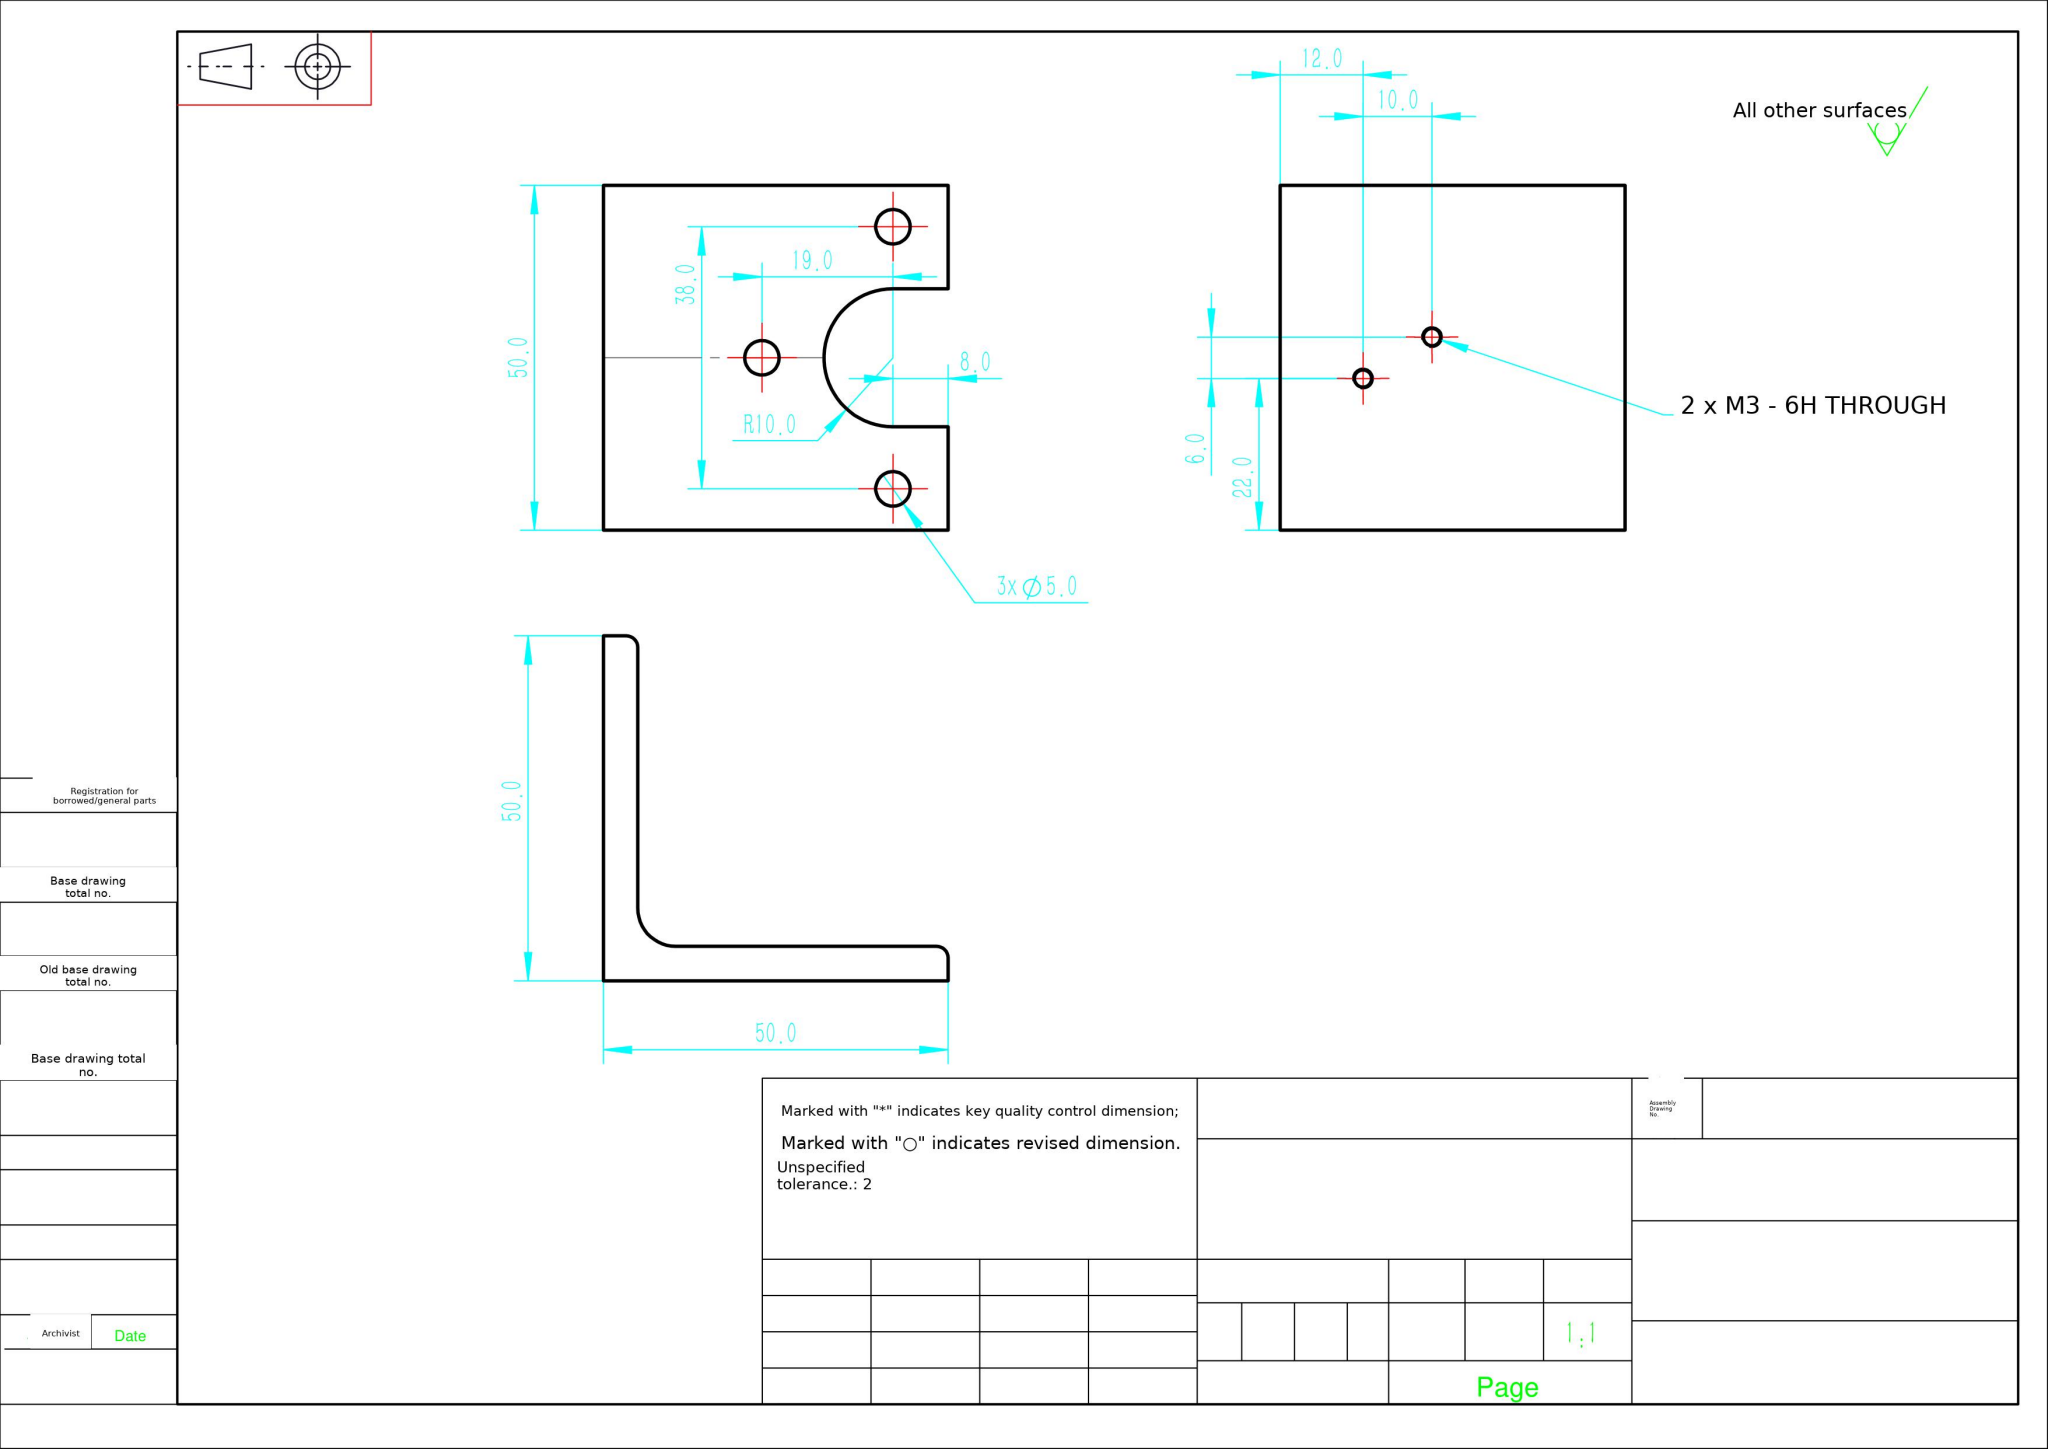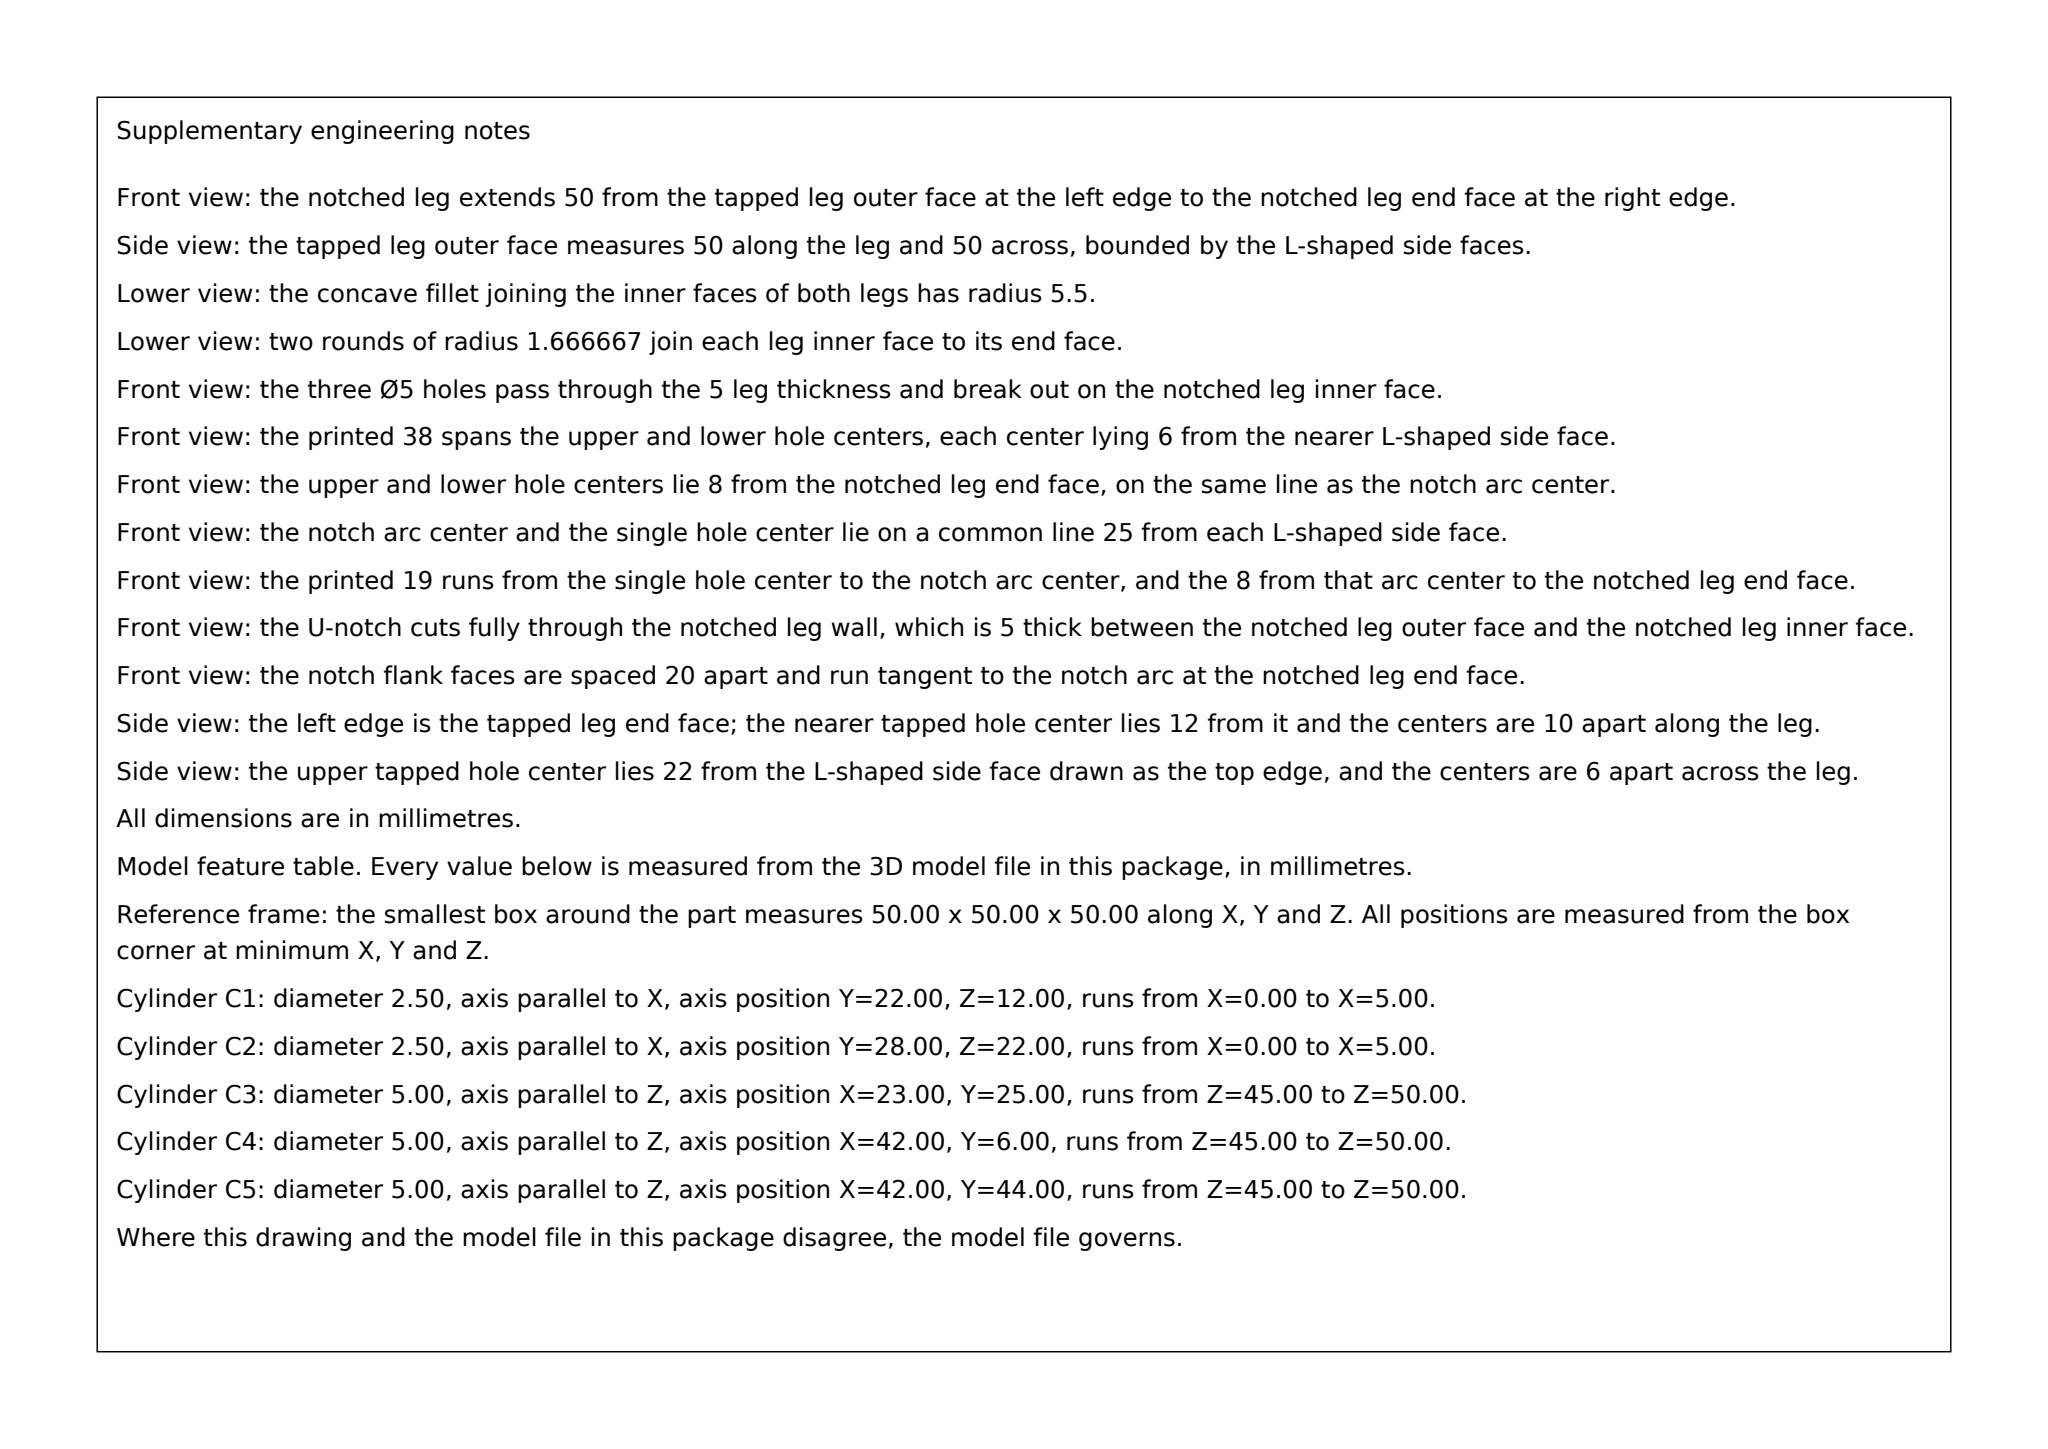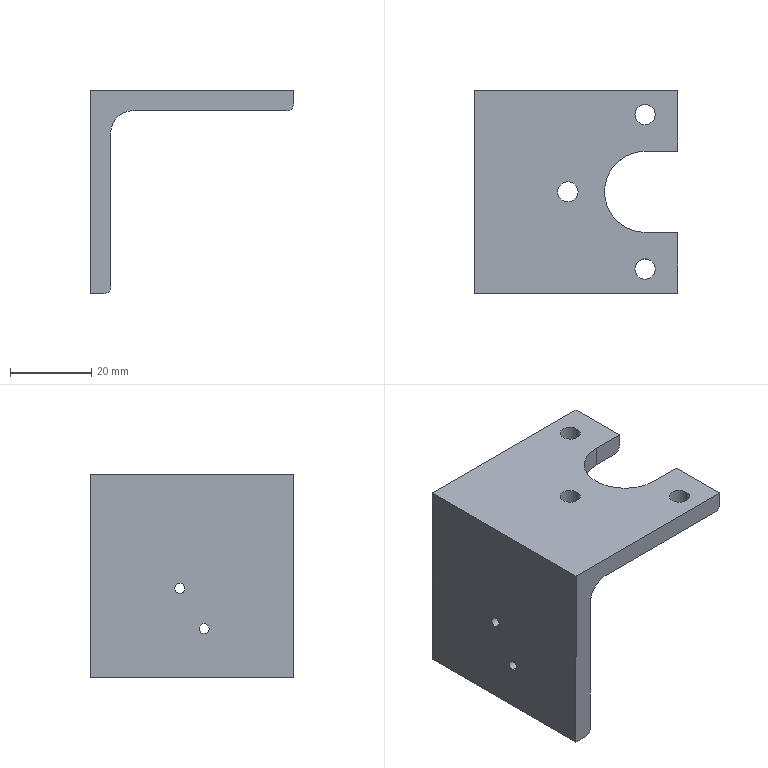Part | SolidWorks | mm | 1 solid | 26 faces | box 50 x 50 x 50 mm | volume 22098 mm3 | cylinder 15 | plane 11 | commonest cylinder face diameters 5 x6 2.5 x4 3.333 x3 11 x1 20 x1
Drawing notes:
HORIZ LEG THK 5.0 (SAME AS VERT LEG) | from the solid: Z planes at 45.0 and 50.0 with bbox Z=50; Ø5 holes axis z length 5.0
build123d program:
from build123d import *

# Parameters (mm, degrees)
STRUCTURAL_MEMBER1_DEPTH = 50
CUT_EXTRUDE1_REACH       = 66.413
SKETCH3_R                = 2.5
M3_TAPPED_HOLE1_D        = 2.5


with BuildPart() as part:
    # Sketch1 → Structural Member1 (new body)
    with BuildSketch(Plane(origin=(-32, -25, 0), x_dir=(1, 0, 0), z_dir=(0, -1, 0))):
        with BuildLine():
            Line((50, 0), (0, 0))
            Line((0, 0), (0, -50))
            Line((0, -50), (3.333, -50))
            ThreePointArc((3.333, -50), (4.512, -49.512), (5, -48.333))
            Line((5, -48.333), (5, -10.5))
            ThreePointArc((5, -10.5), (6.611, -6.611), (10.5, -5))
            Line((10.5, -5), (48.333, -5))
            ThreePointArc((48.333, -5), (49.512, -4.512), (50, -3.333))
            Line((50, -3.333), (50, 0))
        make_face()
    extrude(amount=-STRUCTURAL_MEMBER1_DEPTH)

    # Sketch3 → Cut-Extrude1 (cut, up to next)
    with BuildSketch(Plane.XY, mode=Mode.PRIVATE) as cut_extrude1_sk1:
        with Locations((10, -19)):
            Circle(SKETCH3_R)
    cut_extrude1_tool1 = extrude(cut_extrude1_sk1.sketch, amount=-CUT_EXTRUDE1_REACH, mode=Mode.PRIVATE) & part.part
    # Sketch3 → Cut-Extrude1 (cut, up to next)
    with BuildSketch(Plane.XY, mode=Mode.PRIVATE) as cut_extrude1_sk2:
        with Locations((-9, 0)):
            Circle(SKETCH3_R)
    cut_extrude1_tool2 = extrude(cut_extrude1_sk2.sketch, amount=-CUT_EXTRUDE1_REACH, mode=Mode.PRIVATE) & part.part
    # Sketch3 → Cut-Extrude1 (cut, up to next)
    with BuildSketch(Plane.XY, mode=Mode.PRIVATE) as cut_extrude1_sk3:
        with Locations((10, 19)):
            Circle(SKETCH3_R)
    cut_extrude1_tool3 = extrude(cut_extrude1_sk3.sketch, amount=-CUT_EXTRUDE1_REACH, mode=Mode.PRIVATE) & part.part
    # Sketch3 → Cut-Extrude1 (cut, up to next)
    with BuildSketch(Plane.XY, mode=Mode.PRIVATE) as cut_extrude1_sk4:
        with BuildLine():
            Line((10, 10), (18, 10))
            ThreePointArc((18, 10), (28, 0), (18, -10))
            Line((18, -10), (10, -10))
            ThreePointArc((10, -10), (0, 0), (10, 10))
        make_face()
    cut_extrude1_tool4 = extrude(cut_extrude1_sk4.sketch, amount=-CUT_EXTRUDE1_REACH, mode=Mode.PRIVATE) & part.part
    add(cut_extrude1_tool1.solids().sort_by_distance((10, -19, 0))[0], mode=Mode.SUBTRACT)
    add(cut_extrude1_tool2.solids().sort_by_distance((-9, 0, 0))[0], mode=Mode.SUBTRACT)
    add(cut_extrude1_tool3.solids().sort_by_distance((10, 19, 0))[0], mode=Mode.SUBTRACT)
    add(cut_extrude1_tool4.solids().sort_by_distance((14, 0, 0))[0], mode=Mode.SUBTRACT)

    # M3 Tapped Hole1 (through all)
    with Locations(Plane.ZY.offset(32)):
        with Locations((-28, 3), (-38, -3)):
            Hole(M3_TAPPED_HOLE1_D / 2)


solid = part.part
STEP:
#1=CARTESIAN_POINT('',(-27.,3.,-26.75));
#2=VERTEX_POINT('',#1);
#3=CARTESIAN_POINT('',(-27.,3.,-29.25));
#4=VERTEX_POINT('',#3);
#5=CARTESIAN_POINT('',(-27.,3.,-28.));
#6=DIRECTION('',(1.,0.,-0.));
#7=DIRECTION('',(-0.,0.,-1.));
#8=AXIS2_PLACEMENT_3D('',#5,#6,#7);
#9=CIRCLE('',#8,1.25);
#10=EDGE_CURVE('',#2,#4,#9,.T.);
#11=ORIENTED_EDGE('',*,*,#10,.T.);
#12=CARTESIAN_POINT('',(-32.,3.,-29.25));
#13=VERTEX_POINT('',#12);
#14=CARTESIAN_POINT('',(-32.,3.,-29.25));
#15=DIRECTION('',(-1.,0.,0.));
#16=VECTOR('',#15,1000.);
#17=LINE('',#14,#16);
#18=EDGE_CURVE('',#4,#13,#17,.T.);
#19=ORIENTED_EDGE('',*,*,#18,.T.);
#20=CARTESIAN_POINT('',(-32.,3.,-26.75));
#21=VERTEX_POINT('',#20);
#22=CARTESIAN_POINT('',(-32.,3.,-28.));
#23=DIRECTION('',(-1.,0.,0.));
#24=DIRECTION('',(0.,0.,1.));
#25=AXIS2_PLACEMENT_3D('',#22,#23,#24);
#26=CIRCLE('',#25,1.25);
#27=EDGE_CURVE('',#13,#21,#26,.T.);
#28=ORIENTED_EDGE('',*,*,#27,.T.);
#29=CARTESIAN_POINT('',(-32.,3.,-26.75));
#30=DIRECTION('',(-1.,0.,0.));
#31=VECTOR('',#30,1000.);
#32=LINE('',#29,#31);
#33=EDGE_CURVE('',#2,#21,#32,.T.);
#34=ORIENTED_EDGE('',*,*,#33,.F.);
#35=EDGE_LOOP('',(#11,#19,#28,#34));
#36=FACE_OUTER_BOUND('',#35,.T.);
#37=CARTESIAN_POINT('',(-32.,3.,-28.));
#38=DIRECTION('',(-1.,0.,0.));
#39=DIRECTION('',(0.,0.,1.));
#40=AXIS2_PLACEMENT_3D('',#37,#38,#39);
#41=CYLINDRICAL_SURFACE('',#40,1.25);
#42=ADVANCED_FACE('',(#36),#41,.F.);
#43=CARTESIAN_POINT('',(-27.,-3.,-36.75));
#44=VERTEX_POINT('',#43);
#45=CARTESIAN_POINT('',(-27.,-3.,-39.25));
#46=VERTEX_POINT('',#45);
#47=CARTESIAN_POINT('',(-27.,-3.,-38.));
#48=DIRECTION('',(1.,0.,-0.));
#49=DIRECTION('',(-0.,0.,-1.));
#50=AXIS2_PLACEMENT_3D('',#47,#48,#49);
#51=CIRCLE('',#50,1.25);
#52=EDGE_CURVE('',#44,#46,#51,.T.);
#53=ORIENTED_EDGE('',*,*,#52,.T.);
#54=CARTESIAN_POINT('',(-32.,-3.,-39.25));
#55=VERTEX_POINT('',#54);
#56=CARTESIAN_POINT('',(-32.,-3.,-39.25));
#57=DIRECTION('',(-1.,0.,0.));
#58=VECTOR('',#57,1000.);
#59=LINE('',#56,#58);
#60=EDGE_CURVE('',#46,#55,#59,.T.);
#61=ORIENTED_EDGE('',*,*,#60,.T.);
#62=CARTESIAN_POINT('',(-32.,-3.,-36.75));
#63=VERTEX_POINT('',#62);
#64=CARTESIAN_POINT('',(-32.,-3.,-38.));
#65=DIRECTION('',(-1.,0.,0.));
#66=DIRECTION('',(0.,0.,1.));
#67=AXIS2_PLACEMENT_3D('',#64,#65,#66);
#68=CIRCLE('',#67,1.25);
#69=EDGE_CURVE('',#55,#63,#68,.T.);
#70=ORIENTED_EDGE('',*,*,#69,.T.);
#71=CARTESIAN_POINT('',(-32.,-3.,-36.75));
#72=DIRECTION('',(-1.,0.,0.));
#73=VECTOR('',#72,1000.);
#74=LINE('',#71,#73);
#75=EDGE_CURVE('',#44,#63,#74,.T.);
#76=ORIENTED_EDGE('',*,*,#75,.F.);
#77=EDGE_LOOP('',(#53,#61,#70,#76));
#78=FACE_OUTER_BOUND('',#77,.T.);
#79=CARTESIAN_POINT('',(-32.,-3.,-38.));
#80=DIRECTION('',(-1.,0.,0.));
#81=DIRECTION('',(0.,0.,1.));
#82=AXIS2_PLACEMENT_3D('',#79,#80,#81);
#83=CYLINDRICAL_SURFACE('',#82,1.25);
#84=ADVANCED_FACE('',(#78),#83,.F.);
#85=CARTESIAN_POINT('',(7.5,19.,-5.));
#86=VERTEX_POINT('',#85);
#87=CARTESIAN_POINT('',(12.5,19.,-5.));
#88=VERTEX_POINT('',#87);
#89=CARTESIAN_POINT('',(10.,19.,-5.));
#90=DIRECTION('',(0.,0.,1.));
#91=DIRECTION('',(-1.,0.,0.));
#92=AXIS2_PLACEMENT_3D('',#89,#90,#91);
#93=CIRCLE('',#92,2.5);
#94=EDGE_CURVE('',#86,#88,#93,.T.);
#95=ORIENTED_EDGE('',*,*,#94,.F.);
#96=CARTESIAN_POINT('',(7.5,19.,0.));
#97=VERTEX_POINT('',#96);
#98=CARTESIAN_POINT('',(7.5,19.,-50.001));
#99=DIRECTION('',(0.,0.,1.));
#100=VECTOR('',#99,1000.);
#101=LINE('',#98,#100);
#102=EDGE_CURVE('',#86,#97,#101,.T.);
#103=ORIENTED_EDGE('',*,*,#102,.T.);
#104=CARTESIAN_POINT('',(12.5,19.,0.));
#105=VERTEX_POINT('',#104);
#106=CARTESIAN_POINT('',(10.,19.,0.));
#107=DIRECTION('',(0.,0.,1.));
#108=DIRECTION('',(1.,0.,0.));
#109=AXIS2_PLACEMENT_3D('',#106,#107,#108);
#110=CIRCLE('',#109,2.5);
#111=EDGE_CURVE('',#97,#105,#110,.T.);
#112=ORIENTED_EDGE('',*,*,#111,.T.);
#113=CARTESIAN_POINT('',(12.5,19.,-50.001));
#114=DIRECTION('',(0.,0.,1.));
#115=VECTOR('',#114,1000.);
#116=LINE('',#113,#115);
#117=EDGE_CURVE('',#88,#105,#116,.T.);
#118=ORIENTED_EDGE('',*,*,#117,.F.);
#119=EDGE_LOOP('',(#95,#103,#112,#118));
#120=FACE_OUTER_BOUND('',#119,.T.);
#121=CARTESIAN_POINT('',(10.,19.,-50.001));
#122=DIRECTION('',(0.,0.,1.));
#123=DIRECTION('',(1.,0.,0.));
#124=AXIS2_PLACEMENT_3D('',#121,#122,#123);
#125=CYLINDRICAL_SURFACE('',#124,2.5);
#126=ADVANCED_FACE('',(#120),#125,.F.);
#127=CARTESIAN_POINT('',(-11.5,-0.,-5.));
#128=VERTEX_POINT('',#127);
#129=CARTESIAN_POINT('',(-6.5,-0.,-5.));
#130=VERTEX_POINT('',#129);
#131=CARTESIAN_POINT('',(-9.,-0.,-5.));
#132=DIRECTION('',(0.,0.,1.));
#133=DIRECTION('',(-1.,0.,0.));
#134=AXIS2_PLACEMENT_3D('',#131,#132,#133);
#135=CIRCLE('',#134,2.5);
#136=EDGE_CURVE('',#128,#130,#135,.T.);
#137=ORIENTED_EDGE('',*,*,#136,.F.);
#138=CARTESIAN_POINT('',(-11.5,-0.,0.));
#139=VERTEX_POINT('',#138);
#140=CARTESIAN_POINT('',(-11.5,-0.,-50.001));
#141=DIRECTION('',(0.,0.,1.));
#142=VECTOR('',#141,1000.);
#143=LINE('',#140,#142);
#144=EDGE_CURVE('',#128,#139,#143,.T.);
#145=ORIENTED_EDGE('',*,*,#144,.T.);
#146=CARTESIAN_POINT('',(-6.5,-0.,0.));
#147=VERTEX_POINT('',#146);
#148=CARTESIAN_POINT('',(-9.,-0.,0.));
#149=DIRECTION('',(0.,0.,1.));
#150=DIRECTION('',(1.,0.,0.));
#151=AXIS2_PLACEMENT_3D('',#148,#149,#150);
#152=CIRCLE('',#151,2.5);
#153=EDGE_CURVE('',#139,#147,#152,.T.);
#154=ORIENTED_EDGE('',*,*,#153,.T.);
#155=CARTESIAN_POINT('',(-6.5,-0.,-50.001));
#156=DIRECTION('',(0.,0.,1.));
#157=VECTOR('',#156,1000.);
#158=LINE('',#155,#157);
#159=EDGE_CURVE('',#130,#147,#158,.T.);
#160=ORIENTED_EDGE('',*,*,#159,.F.);
#161=EDGE_LOOP('',(#137,#145,#154,#160));
#162=FACE_OUTER_BOUND('',#161,.T.);
#163=CARTESIAN_POINT('',(-9.,-0.,-50.001));
#164=DIRECTION('',(0.,0.,1.));
#165=DIRECTION('',(1.,0.,0.));
#166=AXIS2_PLACEMENT_3D('',#163,#164,#165);
#167=CYLINDRICAL_SURFACE('',#166,2.5);
#168=ADVANCED_FACE('',(#162),#167,.F.);
#169=CARTESIAN_POINT('',(7.5,-19.,-5.));
#170=VERTEX_POINT('',#169);
#171=CARTESIAN_POINT('',(12.5,-19.,-5.));
#172=VERTEX_POINT('',#171);
#173=CARTESIAN_POINT('',(10.,-19.,-5.));
#174=DIRECTION('',(0.,0.,1.));
#175=DIRECTION('',(-1.,0.,0.));
#176=AXIS2_PLACEMENT_3D('',#173,#174,#175);
#177=CIRCLE('',#176,2.5);
#178=EDGE_CURVE('',#170,#172,#177,.T.);
#179=ORIENTED_EDGE('',*,*,#178,.F.);
#180=CARTESIAN_POINT('',(7.5,-19.,0.));
#181=VERTEX_POINT('',#180);
#182=CARTESIAN_POINT('',(7.5,-19.,-50.001));
#183=DIRECTION('',(0.,0.,1.));
#184=VECTOR('',#183,1000.);
#185=LINE('',#182,#184);
#186=EDGE_CURVE('',#170,#181,#185,.T.);
#187=ORIENTED_EDGE('',*,*,#186,.T.);
#188=CARTESIAN_POINT('',(12.5,-19.,0.));
#189=VERTEX_POINT('',#188);
#190=CARTESIAN_POINT('',(10.,-19.,0.));
#191=DIRECTION('',(0.,0.,1.));
#192=DIRECTION('',(1.,0.,0.));
#193=AXIS2_PLACEMENT_3D('',#190,#191,#192);
#194=CIRCLE('',#193,2.5);
#195=EDGE_CURVE('',#181,#189,#194,.T.);
#196=ORIENTED_EDGE('',*,*,#195,.T.);
#197=CARTESIAN_POINT('',(12.5,-19.,-50.001));
#198=DIRECTION('',(0.,0.,1.));
#199=VECTOR('',#198,1000.);
#200=LINE('',#197,#199);
#201=EDGE_CURVE('',#172,#189,#200,.T.);
#202=ORIENTED_EDGE('',*,*,#201,.F.);
#203=EDGE_LOOP('',(#179,#187,#196,#202));
#204=FACE_OUTER_BOUND('',#203,.T.);
#205=CARTESIAN_POINT('',(10.,-19.,-50.001));
#206=DIRECTION('',(0.,0.,1.));
#207=DIRECTION('',(1.,0.,0.));
#208=AXIS2_PLACEMENT_3D('',#205,#206,#207);
#209=CYLINDRICAL_SURFACE('',#208,2.5);
#210=ADVANCED_FACE('',(#204),#209,.F.);
#211=CARTESIAN_POINT('',(18.,10.,0.));
#212=VERTEX_POINT('',#211);
#213=CARTESIAN_POINT('',(18.,10.,-3.333));
#214=VERTEX_POINT('',#213);
#215=CARTESIAN_POINT('',(18.,10.,-50.001));
#216=DIRECTION('',(0.,0.,-1.));
#217=VECTOR('',#216,1000.);
#218=LINE('',#215,#217);
#219=EDGE_CURVE('',#212,#214,#218,.T.);
#220=ORIENTED_EDGE('',*,*,#219,.T.);
#221=CARTESIAN_POINT('',(18.,25.,-3.333));
#222=VERTEX_POINT('',#221);
#223=CARTESIAN_POINT('',(18.,25.,-3.333));
#224=DIRECTION('',(0.,-1.,0.));
#225=VECTOR('',#224,1000.);
#226=LINE('',#223,#225);
#227=EDGE_CURVE('',#222,#214,#226,.T.);
#228=ORIENTED_EDGE('',*,*,#227,.F.);
#229=CARTESIAN_POINT('',(18.,25.,-0.));
#230=VERTEX_POINT('',#229);
#231=CARTESIAN_POINT('',(18.,25.,-0.));
#232=DIRECTION('',(0.,-0.,1.));
#233=VECTOR('',#232,1000.);
#234=LINE('',#231,#233);
#235=EDGE_CURVE('',#222,#230,#234,.T.);
#236=ORIENTED_EDGE('',*,*,#235,.T.);
#237=CARTESIAN_POINT('',(18.,25.,-0.));
#238=DIRECTION('',(0.,-1.,0.));
#239=VECTOR('',#238,1000.);
#240=LINE('',#237,#239);
#241=EDGE_CURVE('',#230,#212,#240,.T.);
#242=ORIENTED_EDGE('',*,*,#241,.T.);
#243=EDGE_LOOP('',(#220,#228,#236,#242));
#244=FACE_OUTER_BOUND('',#243,.T.);
#245=CARTESIAN_POINT('',(18.,25.,-0.));
#246=DIRECTION('',(1.,0.,-0.));
#247=DIRECTION('',(-0.,0.,-1.));
#248=AXIS2_PLACEMENT_3D('',#245,#246,#247);
#249=PLANE('',#248);
#250=ADVANCED_FACE('',(#244),#249,.T.);
#251=CARTESIAN_POINT('',(16.333,10.,-5.));
#252=VERTEX_POINT('',#251);
#253=CARTESIAN_POINT('',(16.333,10.,-3.333));
#254=DIRECTION('',(0.,1.,0.));
#255=DIRECTION('',(0.,0.,1.));
#256=AXIS2_PLACEMENT_3D('',#253,#254,#255);
#257=CIRCLE('',#256,1.667);
#258=EDGE_CURVE('',#214,#252,#257,.T.);
#259=ORIENTED_EDGE('',*,*,#258,.T.);
#260=CARTESIAN_POINT('',(16.333,25.,-5.));
#261=VERTEX_POINT('',#260);
#262=CARTESIAN_POINT('',(16.333,25.,-5.));
#263=DIRECTION('',(0.,-1.,0.));
#264=VECTOR('',#263,1000.);
#265=LINE('',#262,#264);
#266=EDGE_CURVE('',#261,#252,#265,.T.);
#267=ORIENTED_EDGE('',*,*,#266,.F.);
#268=CARTESIAN_POINT('',(16.333,25.,-3.333));
#269=DIRECTION('',(-0.,-1.,-0.));
#270=DIRECTION('',(-0.,0.,-1.));
#271=AXIS2_PLACEMENT_3D('',#268,#269,#270);
#272=CIRCLE('',#271,1.667);
#273=EDGE_CURVE('',#261,#222,#272,.T.);
#274=ORIENTED_EDGE('',*,*,#273,.T.);
#275=ORIENTED_EDGE('',*,*,#227,.T.);
#276=EDGE_LOOP('',(#259,#267,#274,#275));
#277=FACE_OUTER_BOUND('',#276,.T.);
#278=CARTESIAN_POINT('',(16.333,25.,-3.333));
#279=DIRECTION('',(0.,-1.,0.));
#280=DIRECTION('',(0.,0.,-1.));
#281=AXIS2_PLACEMENT_3D('',#278,#279,#280);
#282=CYLINDRICAL_SURFACE('',#281,1.667);
#283=ADVANCED_FACE('',(#277),#282,.T.);
#284=CARTESIAN_POINT('',(18.,-10.,-3.333));
#285=VERTEX_POINT('',#284);
#286=CARTESIAN_POINT('',(18.,-10.,-0.));
#287=VERTEX_POINT('',#286);
#288=CARTESIAN_POINT('',(18.,-10.,-50.001));
#289=DIRECTION('',(0.,0.,1.));
#290=VECTOR('',#289,1000.);
#291=LINE('',#288,#290);
#292=EDGE_CURVE('',#285,#287,#291,.T.);
#293=ORIENTED_EDGE('',*,*,#292,.T.);
#294=CARTESIAN_POINT('',(18.,-25.,-0.));
#295=VERTEX_POINT('',#294);
#296=CARTESIAN_POINT('',(18.,25.,-0.));
#297=DIRECTION('',(0.,-1.,0.));
#298=VECTOR('',#297,1000.);
#299=LINE('',#296,#298);
#300=EDGE_CURVE('',#287,#295,#299,.T.);
#301=ORIENTED_EDGE('',*,*,#300,.T.);
#302=CARTESIAN_POINT('',(18.,-25.,-3.333));
#303=VERTEX_POINT('',#302);
#304=CARTESIAN_POINT('',(18.,-25.,-0.));
#305=DIRECTION('',(0.,-0.,1.));
#306=VECTOR('',#305,1000.);
#307=LINE('',#304,#306);
#308=EDGE_CURVE('',#303,#295,#307,.T.);
#309=ORIENTED_EDGE('',*,*,#308,.F.);
#310=CARTESIAN_POINT('',(18.,25.,-3.333));
#311=DIRECTION('',(0.,-1.,0.));
#312=VECTOR('',#311,1000.);
#313=LINE('',#310,#312);
#314=EDGE_CURVE('',#285,#303,#313,.T.);
#315=ORIENTED_EDGE('',*,*,#314,.F.);
#316=EDGE_LOOP('',(#293,#301,#309,#315));
#317=FACE_OUTER_BOUND('',#316,.T.);
#318=CARTESIAN_POINT('',(18.,25.,-0.));
#319=DIRECTION('',(1.,0.,-0.));
#320=DIRECTION('',(-0.,0.,-1.));
#321=AXIS2_PLACEMENT_3D('',#318,#319,#320);
#322=PLANE('',#321);
#323=ADVANCED_FACE('',(#317),#322,.T.);
#324=CARTESIAN_POINT('',(16.333,-10.,-5.));
#325=VERTEX_POINT('',#324);
#326=CARTESIAN_POINT('',(16.333,-10.,-3.333));
#327=DIRECTION('',(0.,-1.,0.));
#328=DIRECTION('',(0.,0.,-1.));
#329=AXIS2_PLACEMENT_3D('',#326,#327,#328);
#330=CIRCLE('',#329,1.667);
#331=EDGE_CURVE('',#325,#285,#330,.T.);
#332=ORIENTED_EDGE('',*,*,#331,.T.);
#333=ORIENTED_EDGE('',*,*,#314,.T.);
#334=CARTESIAN_POINT('',(16.333,-25.,-5.));
#335=VERTEX_POINT('',#334);
#336=CARTESIAN_POINT('',(16.333,-25.,-3.333));
#337=DIRECTION('',(-0.,-1.,-0.));
#338=DIRECTION('',(-0.,0.,-1.));
#339=AXIS2_PLACEMENT_3D('',#336,#337,#338);
#340=CIRCLE('',#339,1.667);
#341=EDGE_CURVE('',#335,#303,#340,.T.);
#342=ORIENTED_EDGE('',*,*,#341,.F.);
#343=CARTESIAN_POINT('',(16.333,25.,-5.));
#344=DIRECTION('',(0.,-1.,0.));
#345=VECTOR('',#344,1000.);
#346=LINE('',#343,#345);
#347=EDGE_CURVE('',#325,#335,#346,.T.);
#348=ORIENTED_EDGE('',*,*,#347,.F.);
#349=EDGE_LOOP('',(#332,#333,#342,#348));
#350=FACE_OUTER_BOUND('',#349,.T.);
#351=CARTESIAN_POINT('',(16.333,25.,-3.333));
#352=DIRECTION('',(0.,-1.,0.));
#353=DIRECTION('',(0.,0.,-1.));
#354=AXIS2_PLACEMENT_3D('',#351,#352,#353);
#355=CYLINDRICAL_SURFACE('',#354,1.667);
#356=ADVANCED_FACE('',(#350),#355,.T.);
#357=CARTESIAN_POINT('',(10.,19.,-5.));
#358=DIRECTION('',(0.,0.,1.));
#359=DIRECTION('',(-1.,0.,0.));
#360=AXIS2_PLACEMENT_3D('',#357,#358,#359);
#361=CIRCLE('',#360,2.5);
#362=EDGE_CURVE('',#88,#86,#361,.T.);
#363=ORIENTED_EDGE('',*,*,#362,.T.);
#364=ORIENTED_EDGE('',*,*,#94,.T.);
#365=EDGE_LOOP('',(#363,#364));
#366=FACE_BOUND('',#365,.T.);
#367=CARTESIAN_POINT('',(10.,10.,-5.));
#368=VERTEX_POINT('',#367);
#369=CARTESIAN_POINT('',(10.,10.,-5.));
#370=DIRECTION('',(-1.,0.,0.));
#371=VECTOR('',#370,1000.);
#372=LINE('',#369,#371);
#373=EDGE_CURVE('',#252,#368,#372,.T.);
#374=ORIENTED_EDGE('',*,*,#373,.T.);
#375=CARTESIAN_POINT('',(10.,-10.,-5.));
#376=VERTEX_POINT('',#375);
#377=CARTESIAN_POINT('',(10.,-0.,-5.));
#378=DIRECTION('',(0.,0.,1.));
#379=DIRECTION('',(-1.,0.,0.));
#380=AXIS2_PLACEMENT_3D('',#377,#378,#379);
#381=CIRCLE('',#380,10.);
#382=EDGE_CURVE('',#368,#376,#381,.T.);
#383=ORIENTED_EDGE('',*,*,#382,.T.);
#384=CARTESIAN_POINT('',(10.,-10.,-5.));
#385=DIRECTION('',(1.,0.,-0.));
#386=VECTOR('',#385,1000.);
#387=LINE('',#384,#386);
#388=EDGE_CURVE('',#376,#325,#387,.T.);
#389=ORIENTED_EDGE('',*,*,#388,.T.);
#390=ORIENTED_EDGE('',*,*,#347,.T.);
#391=CARTESIAN_POINT('',(-21.5,-25.,-5.));
#392=VERTEX_POINT('',#391);
#393=CARTESIAN_POINT('',(16.333,-25.,-5.));
#394=DIRECTION('',(1.,-0.,-0.));
#395=VECTOR('',#394,1000.);
#396=LINE('',#393,#395);
#397=EDGE_CURVE('',#392,#335,#396,.T.);
#398=ORIENTED_EDGE('',*,*,#397,.F.);
#399=CARTESIAN_POINT('',(-21.5,25.,-5.));
#400=VERTEX_POINT('',#399);
#401=CARTESIAN_POINT('',(-21.5,25.,-5.));
#402=DIRECTION('',(0.,-1.,0.));
#403=VECTOR('',#402,1000.);
#404=LINE('',#401,#403);
#405=EDGE_CURVE('',#400,#392,#404,.T.);
#406=ORIENTED_EDGE('',*,*,#405,.F.);
#407=CARTESIAN_POINT('',(16.333,25.,-5.));
#408=DIRECTION('',(1.,-0.,-0.));
#409=VECTOR('',#408,1000.);
#410=LINE('',#407,#409);
#411=EDGE_CURVE('',#400,#261,#410,.T.);
#412=ORIENTED_EDGE('',*,*,#411,.T.);
#413=ORIENTED_EDGE('',*,*,#266,.T.);
#414=EDGE_LOOP('',(#374,#383,#389,#390,#398,#406,#412,#413));
#415=FACE_OUTER_BOUND('',#414,.T.);
#416=CARTESIAN_POINT('',(-9.,-0.,-5.));
#417=DIRECTION('',(0.,0.,1.));
#418=DIRECTION('',(-1.,0.,0.));
#419=AXIS2_PLACEMENT_3D('',#416,#417,#418);
#420=CIRCLE('',#419,2.5);
#421=EDGE_CURVE('',#130,#128,#420,.T.);
#422=ORIENTED_EDGE('',*,*,#421,.T.);
#423=ORIENTED_EDGE('',*,*,#136,.T.);
#424=EDGE_LOOP('',(#422,#423));
#425=FACE_BOUND('',#424,.T.);
#426=CARTESIAN_POINT('',(10.,-19.,-5.));
#427=DIRECTION('',(0.,0.,1.));
#428=DIRECTION('',(-1.,0.,0.));
#429=AXIS2_PLACEMENT_3D('',#426,#427,#428);
#430=CIRCLE('',#429,2.5);
#431=EDGE_CURVE('',#172,#170,#430,.T.);
#432=ORIENTED_EDGE('',*,*,#431,.T.);
#433=ORIENTED_EDGE('',*,*,#178,.T.);
#434=EDGE_LOOP('',(#432,#433));
#435=FACE_BOUND('',#434,.T.);
#436=CARTESIAN_POINT('',(16.333,25.,-5.));
#437=DIRECTION('',(-0.,0.,-1.));
#438=DIRECTION('',(-1.,0.,0.));
#439=AXIS2_PLACEMENT_3D('',#436,#437,#438);
#440=PLANE('',#439);
#441=ADVANCED_FACE('',(#366,#415,#425,#435),#440,.T.);
#442=CARTESIAN_POINT('',(-27.,-25.,-10.5));
#443=VERTEX_POINT('',#442);
#444=CARTESIAN_POINT('',(-21.5,-25.,-10.5));
#445=DIRECTION('',(0.,1.,0.));
#446=DIRECTION('',(0.,-0.,1.));
#447=AXIS2_PLACEMENT_3D('',#444,#445,#446);
#448=CIRCLE('',#447,5.5);
#449=EDGE_CURVE('',#443,#392,#448,.T.);
#450=ORIENTED_EDGE('',*,*,#449,.F.);
#451=CARTESIAN_POINT('',(-27.,25.,-10.5));
#452=VERTEX_POINT('',#451);
#453=CARTESIAN_POINT('',(-27.,25.,-10.5));
#454=DIRECTION('',(0.,-1.,0.));
#455=VECTOR('',#454,1000.);
#456=LINE('',#453,#455);
#457=EDGE_CURVE('',#452,#443,#456,.T.);
#458=ORIENTED_EDGE('',*,*,#457,.F.);
#459=CARTESIAN_POINT('',(-21.5,25.,-10.5));
#460=DIRECTION('',(0.,1.,0.));
#461=DIRECTION('',(0.,-0.,1.));
#462=AXIS2_PLACEMENT_3D('',#459,#460,#461);
#463=CIRCLE('',#462,5.5);
#464=EDGE_CURVE('',#452,#400,#463,.T.);
#465=ORIENTED_EDGE('',*,*,#464,.T.);
#466=ORIENTED_EDGE('',*,*,#405,.T.);
#467=EDGE_LOOP('',(#450,#458,#465,#466));
#468=FACE_OUTER_BOUND('',#467,.T.);
#469=CARTESIAN_POINT('',(-21.5,25.,-10.5));
#470=DIRECTION('',(0.,-1.,0.));
#471=DIRECTION('',(0.,0.,-1.));
#472=AXIS2_PLACEMENT_3D('',#469,#470,#471);
#473=CYLINDRICAL_SURFACE('',#472,5.5);
#474=ADVANCED_FACE('',(#468),#473,.F.);
#475=ORIENTED_EDGE('',*,*,#10,.F.);
#476=CARTESIAN_POINT('',(-27.,3.,-28.));
#477=DIRECTION('',(1.,0.,-0.));
#478=DIRECTION('',(-0.,0.,-1.));
#479=AXIS2_PLACEMENT_3D('',#476,#477,#478);
#480=CIRCLE('',#479,1.25);
#481=EDGE_CURVE('',#4,#2,#480,.T.);
#482=ORIENTED_EDGE('',*,*,#481,.F.);
#483=EDGE_LOOP('',(#475,#482));
#484=FACE_BOUND('',#483,.T.);
#485=ORIENTED_EDGE('',*,*,#52,.F.);
#486=CARTESIAN_POINT('',(-27.,-3.,-38.));
#487=DIRECTION('',(1.,0.,-0.));
#488=DIRECTION('',(-0.,0.,-1.));
#489=AXIS2_PLACEMENT_3D('',#486,#487,#488);
#490=CIRCLE('',#489,1.25);
#491=EDGE_CURVE('',#46,#44,#490,.T.);
#492=ORIENTED_EDGE('',*,*,#491,.F.);
#493=EDGE_LOOP('',(#485,#492));
#494=FACE_BOUND('',#493,.T.);
#495=CARTESIAN_POINT('',(-27.,-25.,-48.333));
#496=VERTEX_POINT('',#495);
#497=CARTESIAN_POINT('',(-27.,-25.,-10.5));
#498=DIRECTION('',(0.,-0.,1.));
#499=VECTOR('',#498,1000.);
#500=LINE('',#497,#499);
#501=EDGE_CURVE('',#496,#443,#500,.T.);
#502=ORIENTED_EDGE('',*,*,#501,.F.);
#503=CARTESIAN_POINT('',(-27.,25.,-48.333));
#504=VERTEX_POINT('',#503);
#505=CARTESIAN_POINT('',(-27.,25.,-48.333));
#506=DIRECTION('',(0.,-1.,0.));
#507=VECTOR('',#506,1000.);
#508=LINE('',#505,#507);
#509=EDGE_CURVE('',#504,#496,#508,.T.);
#510=ORIENTED_EDGE('',*,*,#509,.F.);
#511=CARTESIAN_POINT('',(-27.,25.,-10.5));
#512=DIRECTION('',(0.,-0.,1.));
#513=VECTOR('',#512,1000.);
#514=LINE('',#511,#513);
#515=EDGE_CURVE('',#504,#452,#514,.T.);
#516=ORIENTED_EDGE('',*,*,#515,.T.);
#517=ORIENTED_EDGE('',*,*,#457,.T.);
#518=EDGE_LOOP('',(#502,#510,#516,#517));
#519=FACE_OUTER_BOUND('',#518,.T.);
#520=CARTESIAN_POINT('',(-27.,25.,-10.5));
#521=DIRECTION('',(1.,0.,-0.));
#522=DIRECTION('',(-0.,0.,-1.));
#523=AXIS2_PLACEMENT_3D('',#520,#521,#522);
#524=PLANE('',#523);
#525=ADVANCED_FACE('',(#484,#494,#519),#524,.T.);
#526=CARTESIAN_POINT('',(-28.667,-25.,-50.));
#527=VERTEX_POINT('',#526);
#528=CARTESIAN_POINT('',(-28.667,-25.,-48.333));
#529=DIRECTION('',(-0.,-1.,-0.));
#530=DIRECTION('',(0.,-0.,1.));
#531=AXIS2_PLACEMENT_3D('',#528,#529,#530);
#532=CIRCLE('',#531,1.667);
#533=EDGE_CURVE('',#527,#496,#532,.T.);
#534=ORIENTED_EDGE('',*,*,#533,.F.);
#535=CARTESIAN_POINT('',(-28.667,25.,-50.));
#536=VERTEX_POINT('',#535);
#537=CARTESIAN_POINT('',(-28.667,25.,-50.));
#538=DIRECTION('',(0.,-1.,0.));
#539=VECTOR('',#538,1000.);
#540=LINE('',#537,#539);
#541=EDGE_CURVE('',#536,#527,#540,.T.);
#542=ORIENTED_EDGE('',*,*,#541,.F.);
#543=CARTESIAN_POINT('',(-28.667,25.,-48.333));
#544=DIRECTION('',(-0.,-1.,-0.));
#545=DIRECTION('',(0.,-0.,1.));
#546=AXIS2_PLACEMENT_3D('',#543,#544,#545);
#547=CIRCLE('',#546,1.667);
#548=EDGE_CURVE('',#536,#504,#547,.T.);
#549=ORIENTED_EDGE('',*,*,#548,.T.);
#550=ORIENTED_EDGE('',*,*,#509,.T.);
#551=EDGE_LOOP('',(#534,#542,#549,#550));
#552=FACE_OUTER_BOUND('',#551,.T.);
#553=CARTESIAN_POINT('',(-28.667,25.,-48.333));
#554=DIRECTION('',(0.,-1.,0.));
#555=DIRECTION('',(0.,0.,-1.));
#556=AXIS2_PLACEMENT_3D('',#553,#554,#555);
#557=CYLINDRICAL_SURFACE('',#556,1.667);
#558=ADVANCED_FACE('',(#552),#557,.T.);
#559=CARTESIAN_POINT('',(-32.,-25.,-50.));
#560=VERTEX_POINT('',#559);
#561=CARTESIAN_POINT('',(-32.,-25.,-50.));
#562=DIRECTION('',(1.,0.,-0.));
#563=VECTOR('',#562,1000.);
#564=LINE('',#561,#563);
#565=EDGE_CURVE('',#560,#527,#564,.T.);
#566=ORIENTED_EDGE('',*,*,#565,.F.);
#567=CARTESIAN_POINT('',(-32.,25.,-50.));
#568=VERTEX_POINT('',#567);
#569=CARTESIAN_POINT('',(-32.,25.,-50.));
#570=DIRECTION('',(0.,-1.,0.));
#571=VECTOR('',#570,1000.);
#572=LINE('',#569,#571);
#573=EDGE_CURVE('',#568,#560,#572,.T.);
#574=ORIENTED_EDGE('',*,*,#573,.F.);
#575=CARTESIAN_POINT('',(-32.,25.,-50.));
#576=DIRECTION('',(1.,0.,-0.));
#577=VECTOR('',#576,1000.);
#578=LINE('',#575,#577);
#579=EDGE_CURVE('',#568,#536,#578,.T.);
#580=ORIENTED_EDGE('',*,*,#579,.T.);
#581=ORIENTED_EDGE('',*,*,#541,.T.);
#582=EDGE_LOOP('',(#566,#574,#580,#581));
#583=FACE_OUTER_BOUND('',#582,.T.);
#584=CARTESIAN_POINT('',(-32.,25.,-50.));
#585=DIRECTION('',(-0.,0.,-1.));
#586=DIRECTION('',(-1.,0.,0.));
#587=AXIS2_PLACEMENT_3D('',#584,#585,#586);
#588=PLANE('',#587);
#589=ADVANCED_FACE('',(#583),#588,.T.);
#590=CARTESIAN_POINT('',(-32.,3.,-28.));
#591=DIRECTION('',(-1.,0.,0.));
#592=DIRECTION('',(0.,0.,1.));
#593=AXIS2_PLACEMENT_3D('',#590,#591,#592);
#594=CIRCLE('',#593,1.25);
#595=EDGE_CURVE('',#21,#13,#594,.T.);
#596=ORIENTED_EDGE('',*,*,#595,.F.);
#597=ORIENTED_EDGE('',*,*,#27,.F.);
#598=EDGE_LOOP('',(#596,#597));
#599=FACE_BOUND('',#598,.T.);
#600=CARTESIAN_POINT('',(-32.,-3.,-38.));
#601=DIRECTION('',(-1.,0.,0.));
#602=DIRECTION('',(0.,0.,1.));
#603=AXIS2_PLACEMENT_3D('',#600,#601,#602);
#604=CIRCLE('',#603,1.25);
#605=EDGE_CURVE('',#63,#55,#604,.T.);
#606=ORIENTED_EDGE('',*,*,#605,.F.);
#607=ORIENTED_EDGE('',*,*,#69,.F.);
#608=EDGE_LOOP('',(#606,#607));
#609=FACE_BOUND('',#608,.T.);
#610=CARTESIAN_POINT('',(-32.,-25.,0.));
#611=VERTEX_POINT('',#610);
#612=CARTESIAN_POINT('',(-32.,-25.,0.));
#613=DIRECTION('',(-0.,0.,-1.));
#614=VECTOR('',#613,1000.);
#615=LINE('',#612,#614);
#616=EDGE_CURVE('',#611,#560,#615,.T.);
#617=ORIENTED_EDGE('',*,*,#616,.F.);
#618=CARTESIAN_POINT('',(-32.,25.,0.));
#619=VERTEX_POINT('',#618);
#620=CARTESIAN_POINT('',(-32.,25.,0.));
#621=DIRECTION('',(0.,-1.,0.));
#622=VECTOR('',#621,1000.);
#623=LINE('',#620,#622);
#624=EDGE_CURVE('',#619,#611,#623,.T.);
#625=ORIENTED_EDGE('',*,*,#624,.F.);
#626=CARTESIAN_POINT('',(-32.,25.,0.));
#627=DIRECTION('',(-0.,0.,-1.));
#628=VECTOR('',#627,1000.);
#629=LINE('',#626,#628);
#630=EDGE_CURVE('',#619,#568,#629,.T.);
#631=ORIENTED_EDGE('',*,*,#630,.T.);
#632=ORIENTED_EDGE('',*,*,#573,.T.);
#633=EDGE_LOOP('',(#617,#625,#631,#632));
#634=FACE_OUTER_BOUND('',#633,.T.);
#635=CARTESIAN_POINT('',(-32.,25.,0.));
#636=DIRECTION('',(-1.,0.,0.));
#637=DIRECTION('',(0.,0.,1.));
#638=AXIS2_PLACEMENT_3D('',#635,#636,#637);
#639=PLANE('',#638);
#640=ADVANCED_FACE('',(#599,#609,#634),#639,.T.);
#641=CARTESIAN_POINT('',(10.,19.,0.));
#642=DIRECTION('',(0.,0.,1.));
#643=DIRECTION('',(1.,0.,0.));
#644=AXIS2_PLACEMENT_3D('',#641,#642,#643);
#645=CIRCLE('',#644,2.5);
#646=EDGE_CURVE('',#105,#97,#645,.T.);
#647=ORIENTED_EDGE('',*,*,#646,.F.);
#648=ORIENTED_EDGE('',*,*,#111,.F.);
#649=EDGE_LOOP('',(#647,#648));
#650=FACE_BOUND('',#649,.T.);
#651=CARTESIAN_POINT('',(10.,10.,0.));
#652=VERTEX_POINT('',#651);
#653=CARTESIAN_POINT('',(10.,10.,0.));
#654=DIRECTION('',(-1.,0.,0.));
#655=VECTOR('',#654,1000.);
#656=LINE('',#653,#655);
#657=EDGE_CURVE('',#212,#652,#656,.T.);
#658=ORIENTED_EDGE('',*,*,#657,.F.);
#659=ORIENTED_EDGE('',*,*,#241,.F.);
#660=CARTESIAN_POINT('',(18.,25.,-0.));
#661=DIRECTION('',(-1.,0.,0.));
#662=VECTOR('',#661,1000.);
#663=LINE('',#660,#662);
#664=EDGE_CURVE('',#230,#619,#663,.T.);
#665=ORIENTED_EDGE('',*,*,#664,.T.);
#666=ORIENTED_EDGE('',*,*,#624,.T.);
#667=CARTESIAN_POINT('',(18.,-25.,-0.));
#668=DIRECTION('',(-1.,0.,0.));
#669=VECTOR('',#668,1000.);
#670=LINE('',#667,#669);
#671=EDGE_CURVE('',#295,#611,#670,.T.);
#672=ORIENTED_EDGE('',*,*,#671,.F.);
#673=ORIENTED_EDGE('',*,*,#300,.F.);
#674=CARTESIAN_POINT('',(10.,-10.,-0.));
#675=VERTEX_POINT('',#674);
#676=CARTESIAN_POINT('',(10.,-10.,0.));
#677=DIRECTION('',(1.,0.,0.));
#678=VECTOR('',#677,1000.);
#679=LINE('',#676,#678);
#680=EDGE_CURVE('',#675,#287,#679,.T.);
#681=ORIENTED_EDGE('',*,*,#680,.F.);
#682=CARTESIAN_POINT('',(10.,-0.,0.));
#683=DIRECTION('',(0.,0.,1.));
#684=DIRECTION('',(1.,0.,0.));
#685=AXIS2_PLACEMENT_3D('',#682,#683,#684);
#686=CIRCLE('',#685,10.);
#687=EDGE_CURVE('',#652,#675,#686,.T.);
#688=ORIENTED_EDGE('',*,*,#687,.F.);
#689=EDGE_LOOP('',(#658,#659,#665,#666,#672,#673,#681,#688));
#690=FACE_OUTER_BOUND('',#689,.T.);
#691=CARTESIAN_POINT('',(-9.,-0.,0.));
#692=DIRECTION('',(0.,0.,1.));
#693=DIRECTION('',(1.,0.,0.));
#694=AXIS2_PLACEMENT_3D('',#691,#692,#693);
#695=CIRCLE('',#694,2.5);
#696=EDGE_CURVE('',#147,#139,#695,.T.);
#697=ORIENTED_EDGE('',*,*,#696,.F.);
#698=ORIENTED_EDGE('',*,*,#153,.F.);
#699=EDGE_LOOP('',(#697,#698));
#700=FACE_BOUND('',#699,.T.);
#701=CARTESIAN_POINT('',(10.,-19.,0.));
#702=DIRECTION('',(0.,0.,1.));
#703=DIRECTION('',(1.,0.,0.));
#704=AXIS2_PLACEMENT_3D('',#701,#702,#703);
#705=CIRCLE('',#704,2.5);
#706=EDGE_CURVE('',#189,#181,#705,.T.);
#707=ORIENTED_EDGE('',*,*,#706,.F.);
#708=ORIENTED_EDGE('',*,*,#195,.F.);
#709=EDGE_LOOP('',(#707,#708));
#710=FACE_BOUND('',#709,.T.);
#711=CARTESIAN_POINT('',(18.,25.,-0.));
#712=DIRECTION('',(0.,0.,1.));
#713=DIRECTION('',(1.,0.,-0.));
#714=AXIS2_PLACEMENT_3D('',#711,#712,#713);
#715=PLANE('',#714);
#716=ADVANCED_FACE('',(#650,#690,#700,#710),#715,.T.);
#717=ORIENTED_EDGE('',*,*,#235,.F.);
#718=ORIENTED_EDGE('',*,*,#273,.F.);
#719=ORIENTED_EDGE('',*,*,#411,.F.);
#720=ORIENTED_EDGE('',*,*,#464,.F.);
#721=ORIENTED_EDGE('',*,*,#515,.F.);
#722=ORIENTED_EDGE('',*,*,#548,.F.);
#723=ORIENTED_EDGE('',*,*,#579,.F.);
#724=ORIENTED_EDGE('',*,*,#630,.F.);
#725=ORIENTED_EDGE('',*,*,#664,.F.);
#726=EDGE_LOOP('',(#717,#718,#719,#720,#721,#722,#723,#724,#725));
#727=FACE_OUTER_BOUND('',#726,.T.);
#728=CARTESIAN_POINT('',(16.333,25.,-3.333));
#729=DIRECTION('',(0.,1.,0.));
#730=DIRECTION('',(-0.,0.,-1.));
#731=AXIS2_PLACEMENT_3D('',#728,#729,#730);
#732=PLANE('',#731);
#733=ADVANCED_FACE('',(#727),#732,.T.);
#734=ORIENTED_EDGE('',*,*,#308,.T.);
#735=ORIENTED_EDGE('',*,*,#671,.T.);
#736=ORIENTED_EDGE('',*,*,#616,.T.);
#737=ORIENTED_EDGE('',*,*,#565,.T.);
#738=ORIENTED_EDGE('',*,*,#533,.T.);
#739=ORIENTED_EDGE('',*,*,#501,.T.);
#740=ORIENTED_EDGE('',*,*,#449,.T.);
#741=ORIENTED_EDGE('',*,*,#397,.T.);
#742=ORIENTED_EDGE('',*,*,#341,.T.);
#743=EDGE_LOOP('',(#734,#735,#736,#737,#738,#739,#740,#741,#742));
#744=FACE_OUTER_BOUND('',#743,.T.);
#745=CARTESIAN_POINT('',(16.333,-25.,-3.333));
#746=DIRECTION('',(0.,1.,0.));
#747=DIRECTION('',(-0.,0.,-1.));
#748=AXIS2_PLACEMENT_3D('',#745,#746,#747);
#749=PLANE('',#748);
#750=ADVANCED_FACE('',(#744),#749,.F.);
#751=ORIENTED_EDGE('',*,*,#186,.F.);
#752=ORIENTED_EDGE('',*,*,#431,.F.);
#753=ORIENTED_EDGE('',*,*,#201,.T.);
#754=ORIENTED_EDGE('',*,*,#706,.T.);
#755=EDGE_LOOP('',(#751,#752,#753,#754));
#756=FACE_OUTER_BOUND('',#755,.T.);
#757=CARTESIAN_POINT('',(10.,-19.,-50.001));
#758=DIRECTION('',(0.,0.,1.));
#759=DIRECTION('',(1.,0.,0.));
#760=AXIS2_PLACEMENT_3D('',#757,#758,#759);
#761=CYLINDRICAL_SURFACE('',#760,2.5);
#762=ADVANCED_FACE('',(#756),#761,.F.);
#763=ORIENTED_EDGE('',*,*,#144,.F.);
#764=ORIENTED_EDGE('',*,*,#421,.F.);
#765=ORIENTED_EDGE('',*,*,#159,.T.);
#766=ORIENTED_EDGE('',*,*,#696,.T.);
#767=EDGE_LOOP('',(#763,#764,#765,#766));
#768=FACE_OUTER_BOUND('',#767,.T.);
#769=CARTESIAN_POINT('',(-9.,-0.,-50.001));
#770=DIRECTION('',(0.,0.,1.));
#771=DIRECTION('',(1.,0.,0.));
#772=AXIS2_PLACEMENT_3D('',#769,#770,#771);
#773=CYLINDRICAL_SURFACE('',#772,2.5);
#774=ADVANCED_FACE('',(#768),#773,.F.);
#775=CARTESIAN_POINT('',(10.,10.,-50.001));
#776=DIRECTION('',(0.,0.,1.));
#777=VECTOR('',#776,1000.);
#778=LINE('',#775,#777);
#779=EDGE_CURVE('',#368,#652,#778,.T.);
#780=ORIENTED_EDGE('',*,*,#779,.T.);
#781=ORIENTED_EDGE('',*,*,#687,.T.);
#782=CARTESIAN_POINT('',(10.,-10.,-50.001));
#783=DIRECTION('',(0.,0.,1.));
#784=VECTOR('',#783,1000.);
#785=LINE('',#782,#784);
#786=EDGE_CURVE('',#376,#675,#785,.T.);
#787=ORIENTED_EDGE('',*,*,#786,.F.);
#788=ORIENTED_EDGE('',*,*,#382,.F.);
#789=EDGE_LOOP('',(#780,#781,#787,#788));
#790=FACE_OUTER_BOUND('',#789,.T.);
#791=CARTESIAN_POINT('',(10.,-0.,-50.001));
#792=DIRECTION('',(0.,0.,1.));
#793=DIRECTION('',(1.,0.,0.));
#794=AXIS2_PLACEMENT_3D('',#791,#792,#793);
#795=CYLINDRICAL_SURFACE('',#794,10.);
#796=ADVANCED_FACE('',(#790),#795,.F.);
#797=ORIENTED_EDGE('',*,*,#219,.F.);
#798=ORIENTED_EDGE('',*,*,#657,.T.);
#799=ORIENTED_EDGE('',*,*,#779,.F.);
#800=ORIENTED_EDGE('',*,*,#373,.F.);
#801=ORIENTED_EDGE('',*,*,#258,.F.);
#802=EDGE_LOOP('',(#797,#798,#799,#800,#801));
#803=FACE_OUTER_BOUND('',#802,.T.);
#804=CARTESIAN_POINT('',(10.,10.,-50.001));
#805=DIRECTION('',(0.,1.,0.));
#806=DIRECTION('',(0.,0.,1.));
#807=AXIS2_PLACEMENT_3D('',#804,#805,#806);
#808=PLANE('',#807);
#809=ADVANCED_FACE('',(#803),#808,.F.);
#810=ORIENTED_EDGE('',*,*,#388,.F.);
#811=ORIENTED_EDGE('',*,*,#786,.T.);
#812=ORIENTED_EDGE('',*,*,#680,.T.);
#813=ORIENTED_EDGE('',*,*,#292,.F.);
#814=ORIENTED_EDGE('',*,*,#331,.F.);
#815=EDGE_LOOP('',(#810,#811,#812,#813,#814));
#816=FACE_OUTER_BOUND('',#815,.T.);
#817=CARTESIAN_POINT('',(10.,-10.,-50.001));
#818=DIRECTION('',(0.,-1.,0.));
#819=DIRECTION('',(0.,0.,-1.));
#820=AXIS2_PLACEMENT_3D('',#817,#818,#819);
#821=PLANE('',#820);
#822=ADVANCED_FACE('',(#816),#821,.F.);
#823=ORIENTED_EDGE('',*,*,#102,.F.);
#824=ORIENTED_EDGE('',*,*,#362,.F.);
#825=ORIENTED_EDGE('',*,*,#117,.T.);
#826=ORIENTED_EDGE('',*,*,#646,.T.);
#827=EDGE_LOOP('',(#823,#824,#825,#826));
#828=FACE_OUTER_BOUND('',#827,.T.);
#829=CARTESIAN_POINT('',(10.,19.,-50.001));
#830=DIRECTION('',(0.,0.,1.));
#831=DIRECTION('',(1.,0.,0.));
#832=AXIS2_PLACEMENT_3D('',#829,#830,#831);
#833=CYLINDRICAL_SURFACE('',#832,2.5);
#834=ADVANCED_FACE('',(#828),#833,.F.);
#835=ORIENTED_EDGE('',*,*,#60,.F.);
#836=ORIENTED_EDGE('',*,*,#491,.T.);
#837=ORIENTED_EDGE('',*,*,#75,.T.);
#838=ORIENTED_EDGE('',*,*,#605,.T.);
#839=EDGE_LOOP('',(#835,#836,#837,#838));
#840=FACE_OUTER_BOUND('',#839,.T.);
#841=CARTESIAN_POINT('',(-32.,-3.,-38.));
#842=DIRECTION('',(-1.,0.,0.));
#843=DIRECTION('',(0.,0.,1.));
#844=AXIS2_PLACEMENT_3D('',#841,#842,#843);
#845=CYLINDRICAL_SURFACE('',#844,1.25);
#846=ADVANCED_FACE('',(#840),#845,.F.);
#847=ORIENTED_EDGE('',*,*,#18,.F.);
#848=ORIENTED_EDGE('',*,*,#481,.T.);
#849=ORIENTED_EDGE('',*,*,#33,.T.);
#850=ORIENTED_EDGE('',*,*,#595,.T.);
#851=EDGE_LOOP('',(#847,#848,#849,#850));
#852=FACE_OUTER_BOUND('',#851,.T.);
#853=CARTESIAN_POINT('',(-32.,3.,-28.));
#854=DIRECTION('',(-1.,0.,0.));
#855=DIRECTION('',(0.,0.,1.));
#856=AXIS2_PLACEMENT_3D('',#853,#854,#855);
#857=CYLINDRICAL_SURFACE('',#856,1.25);
#858=ADVANCED_FACE('',(#852),#857,.F.);
#859=CLOSED_SHELL('',(#42,#84,#126,#168,#210,#250,#283,#323,#356,#441,#474,#525,#558,#589,#640,#716,#733,#750,#762,#774,#796,#809,#822,#834,#846,#858));
#860=MANIFOLD_SOLID_BREP('',#859);
#861=CARTESIAN_POINT('',(0.,0.,0.));
#862=DIRECTION('',(0.,0.,1.));
#863=DIRECTION('',(1.,0.,0.));
#864=AXIS2_PLACEMENT_3D('',#861,#862,#863);
#865=(LENGTH_UNIT()NAMED_UNIT(*)SI_UNIT(.MILLI.,.METRE.));
#866=UNCERTAINTY_MEASURE_WITH_UNIT(LENGTH_MEASURE(0.00001),#865,'','');
#867=(NAMED_UNIT(*)PLANE_ANGLE_UNIT()SI_UNIT($,.RADIAN.));
#868=(NAMED_UNIT(*)SI_UNIT($,.STERADIAN.)SOLID_ANGLE_UNIT());
#869=(GEOMETRIC_REPRESENTATION_CONTEXT(3)GLOBAL_UNCERTAINTY_ASSIGNED_CONTEXT((#866))GLOBAL_UNIT_ASSIGNED_CONTEXT((#865,#867,#868))REPRESENTATION_CONTEXT('',''));
#870=ADVANCED_BREP_SHAPE_REPRESENTATION('',(#860,#864),#869);